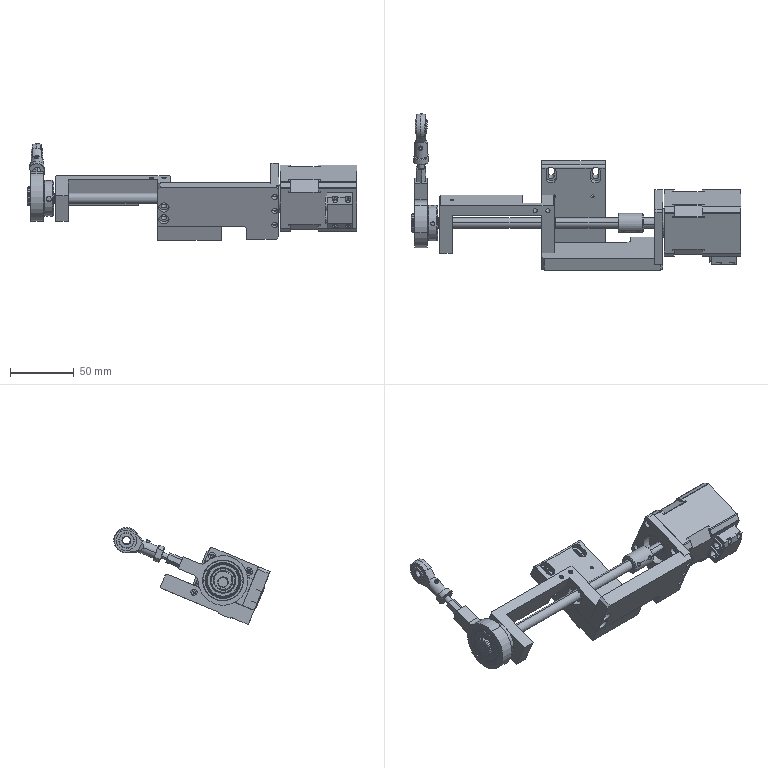Assembly | SolidWorks | mm | 14 component files | 14 solids | 603 faces | box 258.05 x 122.71 x 76.03 mm | volume 249360 mm3 | cylinder 248 | plane 194 | cone 107 | spline 36 | torus 16 | sphere 2 | commonest cylinder face diameters 8 x28 3.3 x28 2 x22 2.5 x14 4.5 x14 15 x12 6 x11 4 x8
Bill of materials:
04-001Screw | 1 |  | Straight cylindrical rod with an integral hexagonal collar at its middle. Equal plain round sections extend from both sides of the hex.
04-003DriveShaft | 1 |  | Long, thin, solid round rod of constant diameter. Two circumferential seam lines split it into three segments.
04-004CouplingSleeve | 1 |  | Thick-walled cylindrical sleeve with a coaxial through bore and chamfered outer end edges. It has four radial holes: two at each end, set at two axial positions.
04-005A1MotorConnectionPlate | 1 | A3 | Rectangular block-like plate. One end has two counterbored slots, and the plate also has two small holes and two larger round holes. A through hole runs in from one side face, and one long edge has a stepped notch.
04-006BottomPlate | 1 |  | Elongated, roughly L-shaped plate. Its outline steps down at one end and has a raised tab or step, with chamfered corners. One end has two counterbored holes and the other end has three holes.
04-007BearingHousing | 1 |  | U-shaped bracket: a bridging beam with two legs. Each leg has a large, aligned through bore. Small holes are drilled in the top and end faces, and the top edge has a rectangular notch.
42mmHybridStepperMotor | 1 |  | Boxy, roughly square-section body with chamfered corners. A cylindrical shaft sticks out from a round pilot boss on one face, and a side-mounted rectangular block has slots and holes. It has recessed bands around the body and two corner holes on the end face.
Bearing6002Z | 1 | 45 | Annular part made of an outer ring and an inner ring, separated by a recessed annular gap on the face. It has a central through bore.
Bearing619-8 | 2 |  | Solid annular ring with a central through bore and rounded outer and inner edges.
ConnectingRod | 1 | 6061 Alloy | Thin-walled ring with an integral straight radial arm or tab, joined to the ring with fillets. The end face of the tab has a hole.
CuttingInductionSeat16-1 | 1 | A3 | Square flat plate with a large central circular hole and four through holes near the corners. One edge face has three holes, and at least two corners are rounded.
EccentricWheel | 1 | GCr15 | Flanged cylindrical hub: a wide disc flange with chamfered edges and a smaller coaxial boss with a groove near its end. A central through bore runs through it, and the flange rim has radial holes.
F-M6X100U | 1 |  | Eye-and-shank part, similar in form to a female rod end: a rounded eye head with a through bore and a raised inner ring held in its face, joined to a cylindrical shank that ends in a hexagonal flange with a blind or through axial bore. A small cylindrical boss with a small center hole sticks out from the side of the shank near the head.
Mates:
1. concentric | 04-001Screw-1 face at (5.226, 51.836, 105.673) dir (0, -0.9233, -0.384) r 2.45 | F-M6X100U-1 face at (5.226, 42.603, 101.833) dir (0, 0.9233, 0.384) r 2.458
2. distance | F-M6X100U-1 face at (-0.7682, 42.701, 101.597) dir (0, -0.9233, -0.384) | 04-001Screw-1 face at (5.226, 37.986, 99.913) dir (0, 0.9233, 0.384)
3. concentric | Bearing6002Z-1 face at (9.426, -5.409, 81.863) dir (-1, 0, 0) r 16 | ConnectingRod-1 face at (0.2264, -5.409, 81.863) dir (1, 0, 0) r 16
4. width | ConnectingRod-1 face at (10.226, -5.409, 81.863) dir (1, 0, 0) | ConnectingRod-1 face at (0.2264, -5.409, 81.863) dir (-1, 0, 0) | Bearing6002Z-1 face at (0.7264, -5.409, 66.163) dir (-1, 0, 0) | Bearing6002Z-1 face at (9.726, -5.409, 68.613) dir (1, 0, 0)
5. concentric | 04-001Screw-1 face at (5.226, 13.98, 89.927) dir (0, 0.9233, 0.384) r 2.45 | ConnectingRod-1 face at (5.226, 27.83, 95.688) dir (0, 0.9233, 0.384) r 2.5
6. coincident | 04-001Screw-1 face at (5.226, 27.83, 95.688) dir (0, -0.9233, -0.384) | ConnectingRod-1 face at (30.911, 29.75, 91.071) dir (0, 0.9233, 0.384)
7. concentric | 04-003DriveShaft-1 face at (169.726, -5.336, 80.465) dir (-1, 0, 0) r 4 | EccentricWheel-1 face at (18.226, -5.336, 80.465) dir (1, 0, 0) r 4
8. concentric | 04-003DriveShaft-1 face at (169.726, -5.336, 80.465) dir (-1, 0, 0) r 4 | EccentricWheel-1 face at (18.226, -5.336, 80.465) dir (1, 0, 0) r 4
9. coincident | 04-003DriveShaft-1 face at (-2.274, -5.336, 80.465) dir (-1, 0, 0) | EccentricWheel-1 face at (-2.274, -5.409, 81.863) dir (-1, 0, 0)
10. concentric | 04-003DriveShaft-1 face at (169.726, -5.336, 80.465) dir (-1, 0, 0) r 4 | Bearing619-8-2 face at (19.726, -5.336, 80.465) dir (1, 0, 0) r 4
11. concentric | 04-003DriveShaft-1 face at (169.726, -5.336, 80.465) dir (-1, 0, 0) r 4 | 04-004CouplingSleeve-1 face at (159.726, -5.336, 80.465) dir (1, 0, 0) r 4
12. coincident | 04-005A1MotorConnectionPlate-2 face at (99.726, 39.515, 87.206) dir (0, -0.384, 0.9233) | 04-006BottomPlate-1 face at (194.726, -29.734, 58.403) dir (0, 0.384, -0.9233)
13. coincident | 04-005A1MotorConnectionPlate-2 face at (99.726, 44.123, 76.126) dir (-1, 0, 0) | 04-006BottomPlate-1 face at (99.726, -42.407, 88.872) dir (-1, 0, 0)
14. coincident | 04-005A1MotorConnectionPlate-2 face at (84.726, -35.303, 71.791) dir (0, -0.9233, -0.384) | 04-006BottomPlate-1 face at (194.726, -42.407, 88.872) dir (0, -0.9233, -0.384)
15. distance | 04-004CouplingSleeve-1 face at (179.726, -5.336, 80.465) dir (1, 0, 0) | 04-003DriveShaft-1 face at (169.726, -5.336, 80.465) dir (1, 0, 0)
16. coincident | Bearing6002Z-1 face at (9.726, -5.409, 74.063) dir (1, 0, 0) | EccentricWheel-1 face at (9.726, -5.409, 81.863) dir (-1, 0, 0)
17. coincident | 04-003DriveShaft-1 face at (19.726, -5.044, 84.454) dir (-1, 0, 0) | Bearing619-8-2 face at (19.726, -5.336, 80.465) dir (-1, 0, 0)
18. coincident | 04-006BottomPlate-1 face at (194.726, -42.407, 88.872) dir (1, 0, 0) | CuttingInductionSeat16-1-2 face at (194.726, -55.893, 133.534) dir (1, 0, 0)
19. coincident | 04-006BottomPlate-1 face at (194.726, -38.068, 90.677) dir (0, 0.9233, 0.384) | CuttingInductionSeat16-1-2 face at (233.526, -21.17, 50.051) dir (0, -0.9233, -0.384)
20. concentric | 42mmHybridStepperMotor-1 face at (193.474, -5.336, 80.465) dir (1, 0, 0) r 11 | CuttingInductionSeat16-1-2 face at (233.526, -5.336, 80.465) dir (-1, 0, 0) r 12.5
21. concentric | 04-004CouplingSleeve-1 face at (159.726, -5.336, 80.465) dir (1, 0, 0) r 4 | 42mmHybridStepperMotor-1 face at (175.474, -5.336, 80.465) dir (1, 0, 0) r 4
22. concentric | 04-006BottomPlate-1 face at (104.726, -32.038, 63.943) dir (0, -0.9233, -0.384) r 4 | 04-007BearingHousing-4 face at (104.726, -22.805, 67.783) dir (0, -0.9233, -0.384) r 1.65
23. concentric | 04-006BottomPlate-1 face at (104.726, -35.879, 73.176) dir (0, -0.9233, -0.384) r 4 | 04-007BearingHousing-4 face at (104.726, -26.645, 77.016) dir (0, -0.9233, -0.384) r 1.65
24. coincident | 04-006BottomPlate-1 face at (194.726, -33.174, 92.713) dir (0, 0.9233, 0.384) | 04-007BearingHousing-4 face at (19.726, -20.501, 62.243) dir (0, -0.9233, -0.384)
25. concentric | Bearing6002Z-1 face at (9.426, -5.409, 81.863) dir (-1, 0, 0) r 7.5 | EccentricWheel-1 face at (-2.274, -5.409, 81.863) dir (1, 0, 0) r 7.5